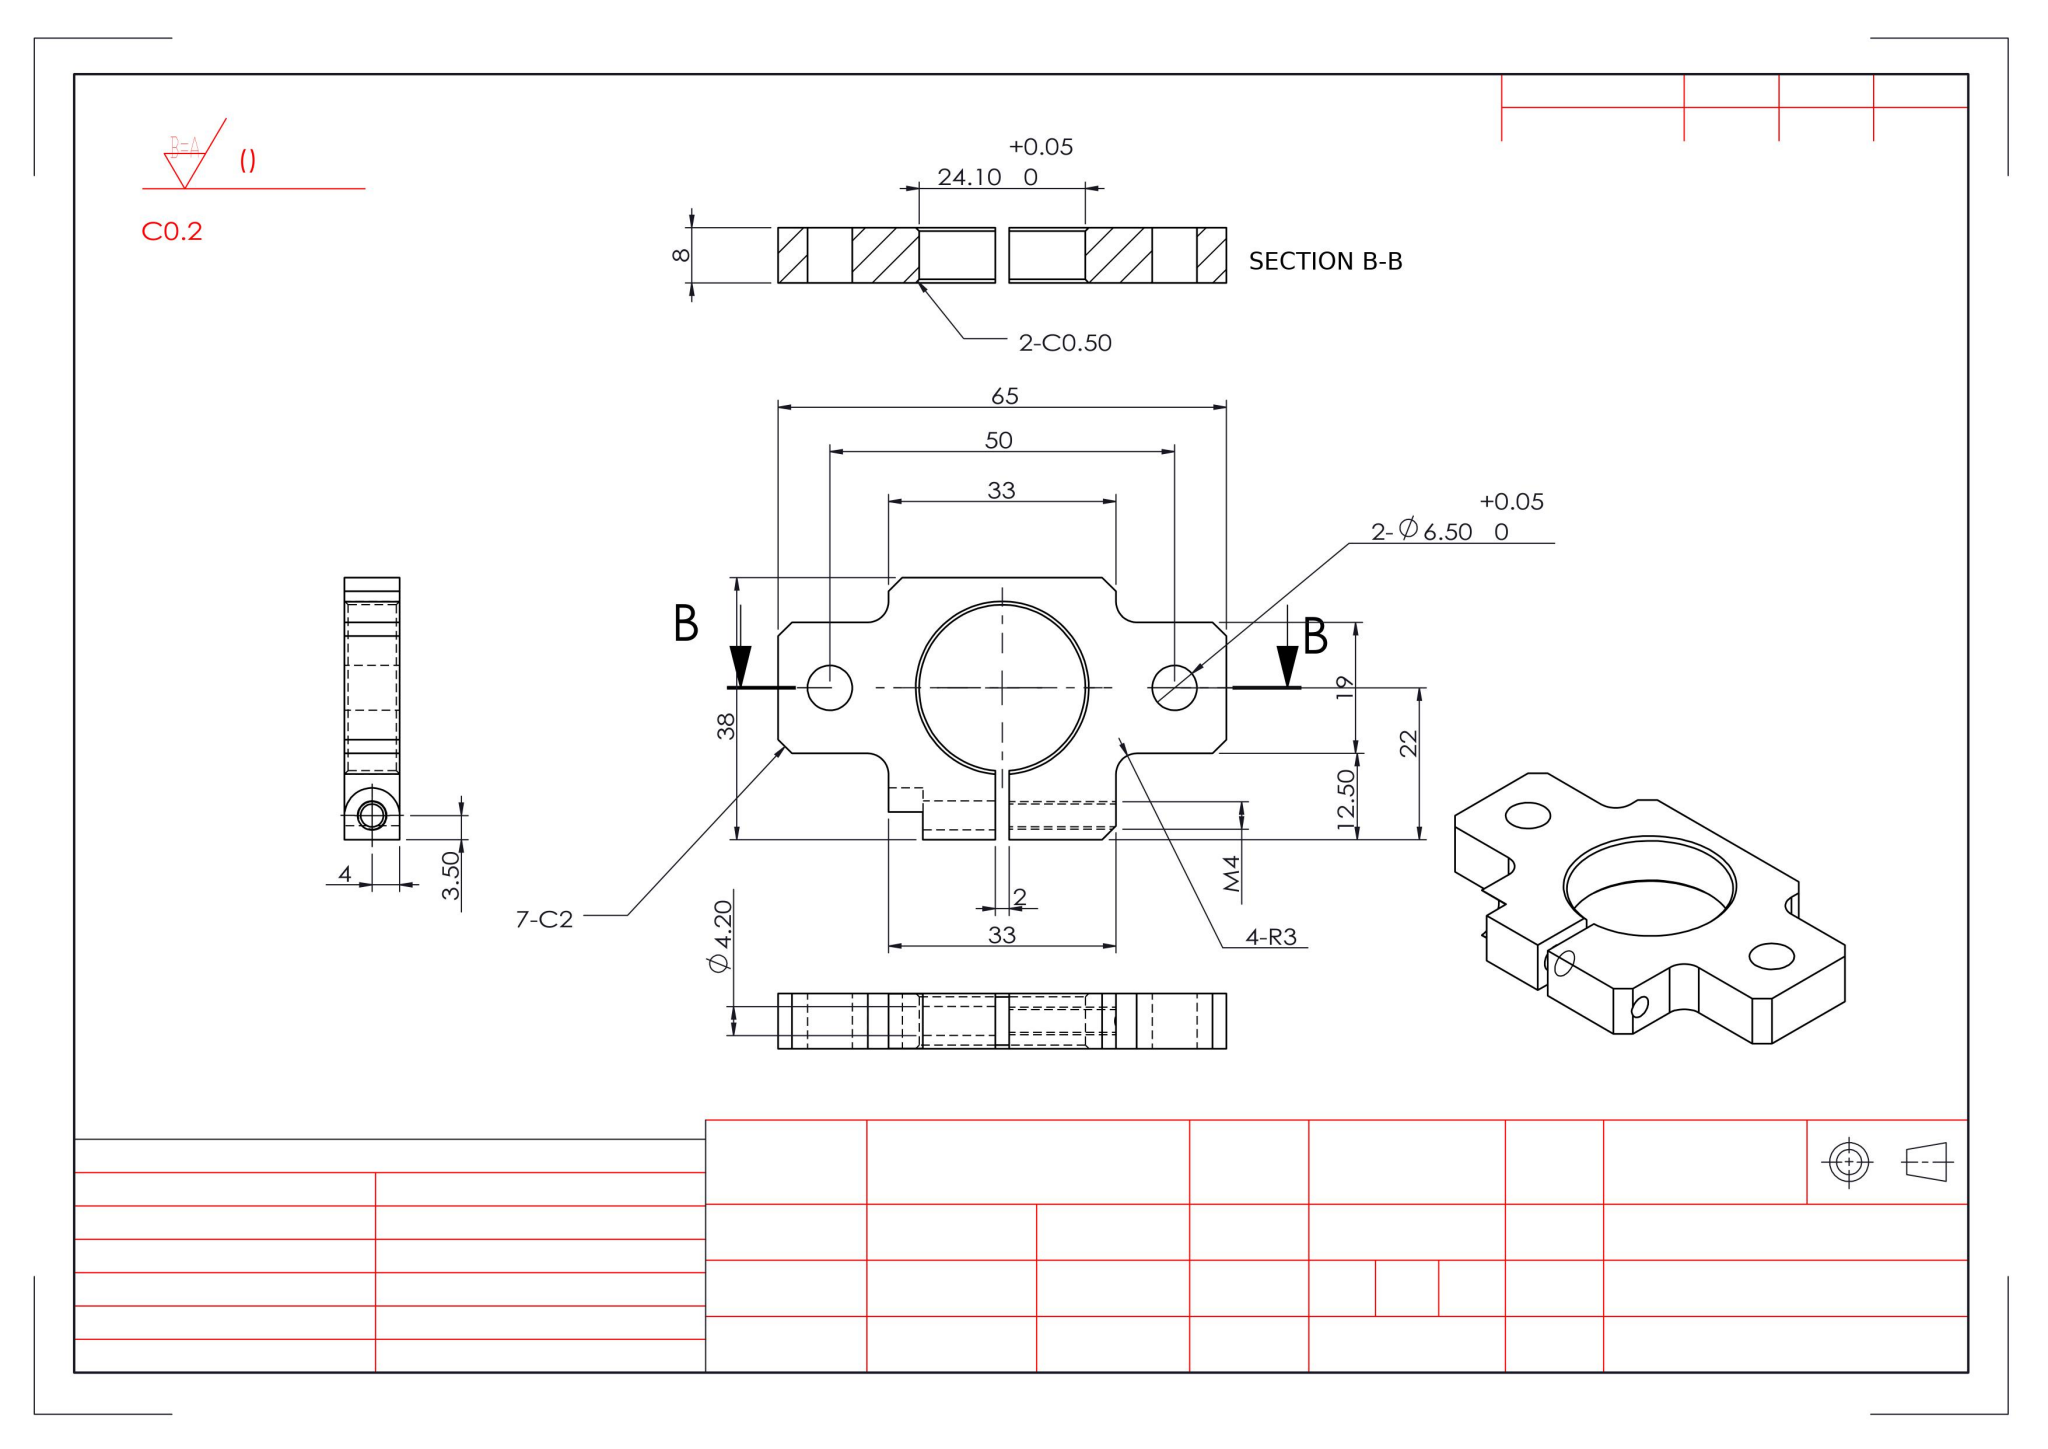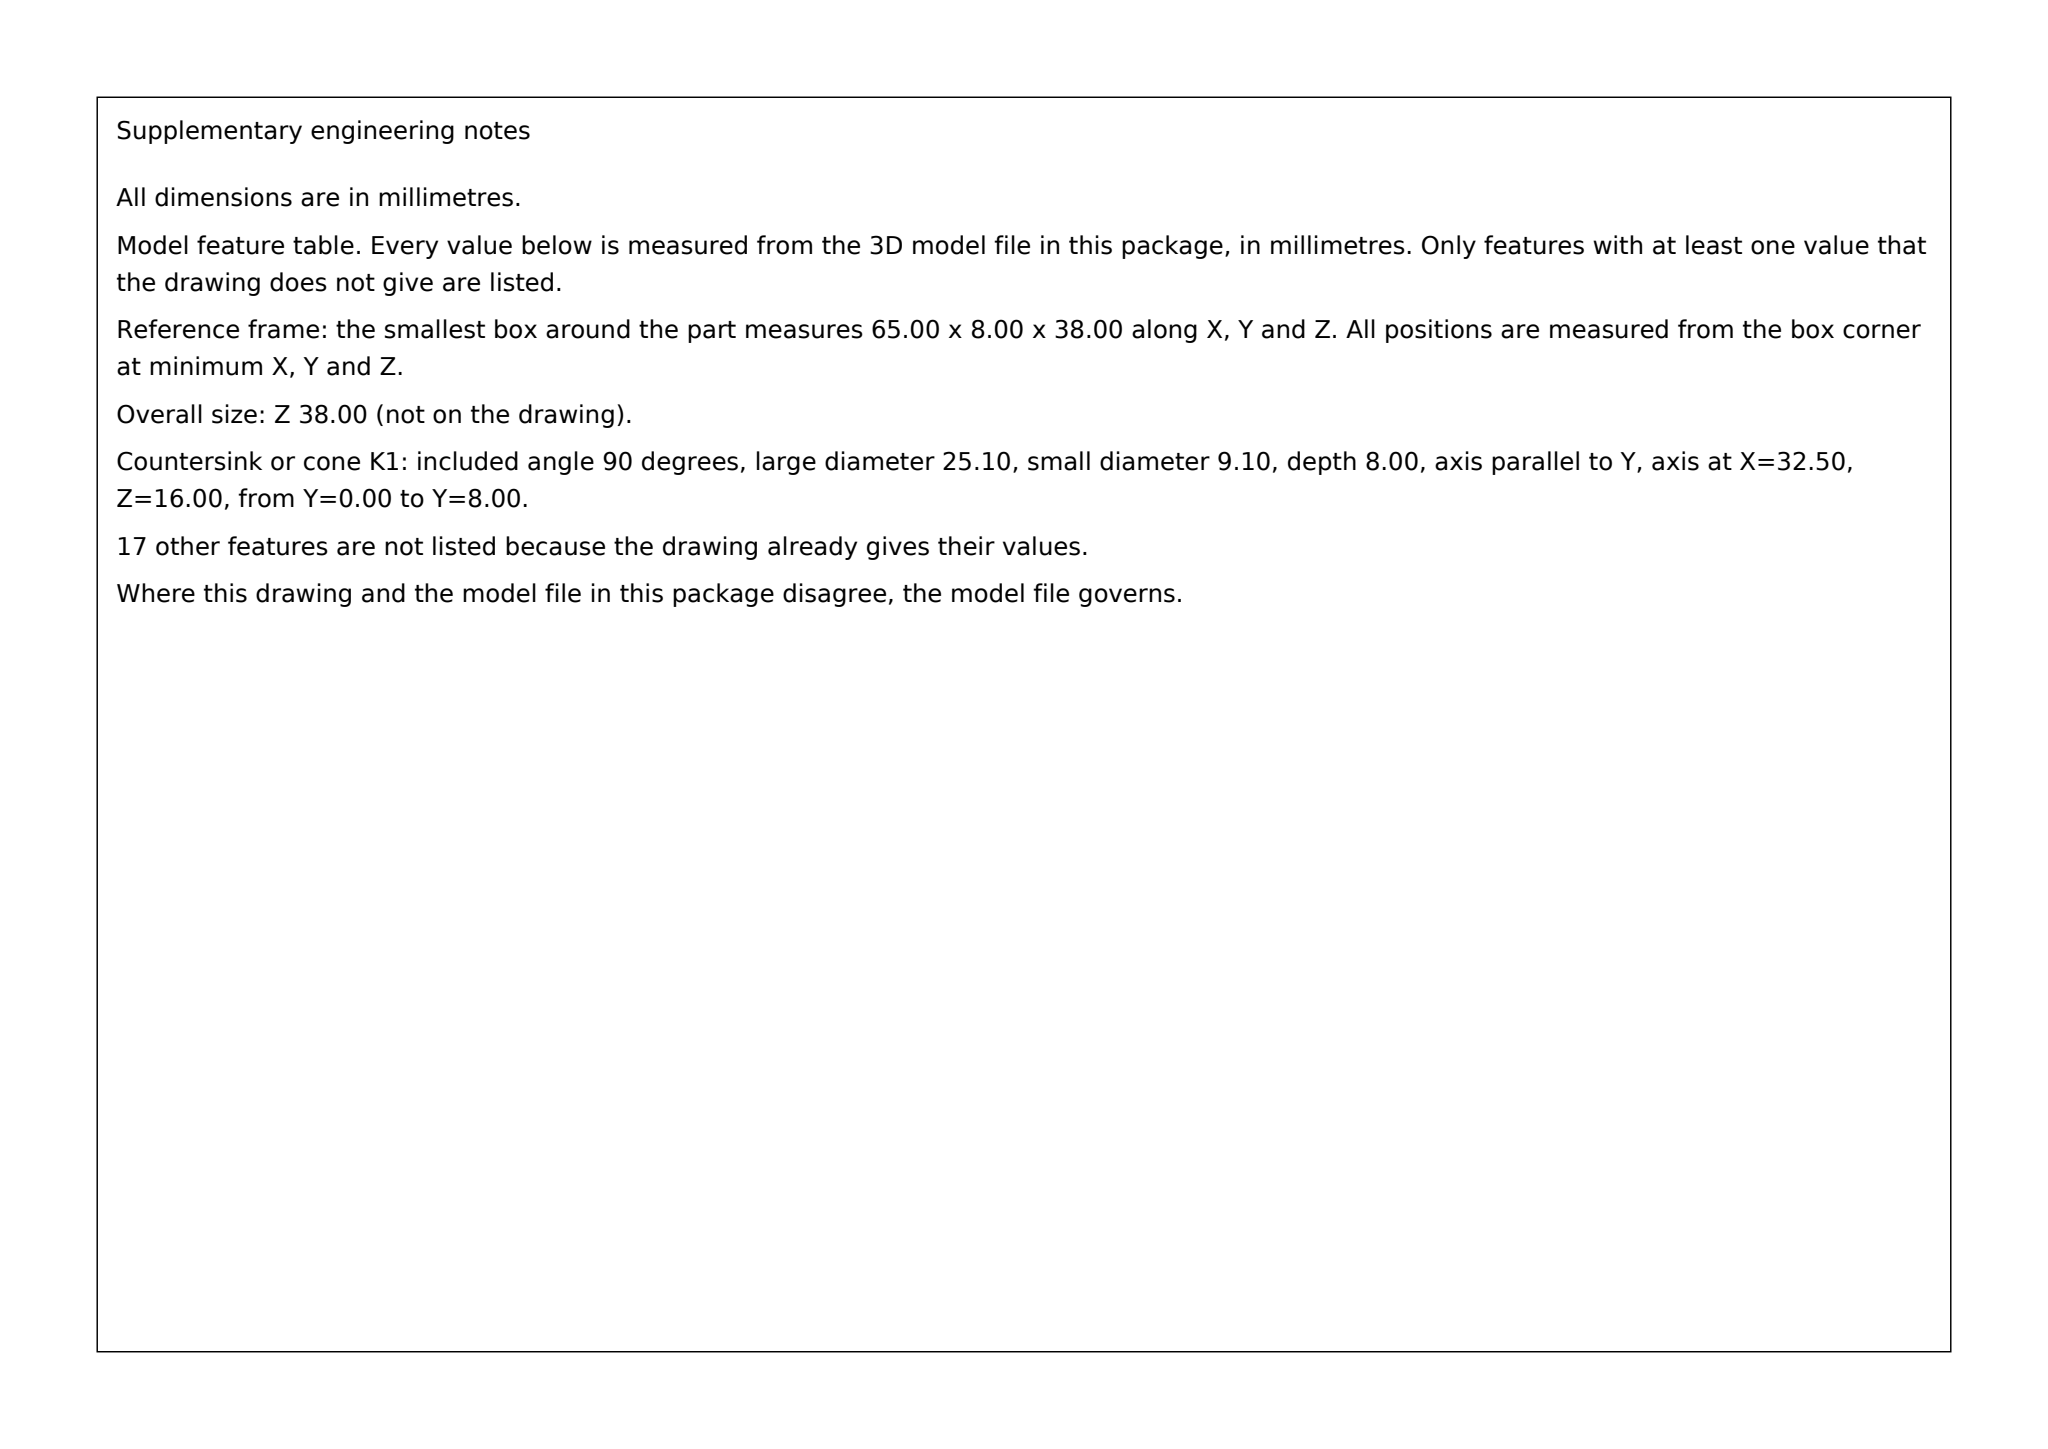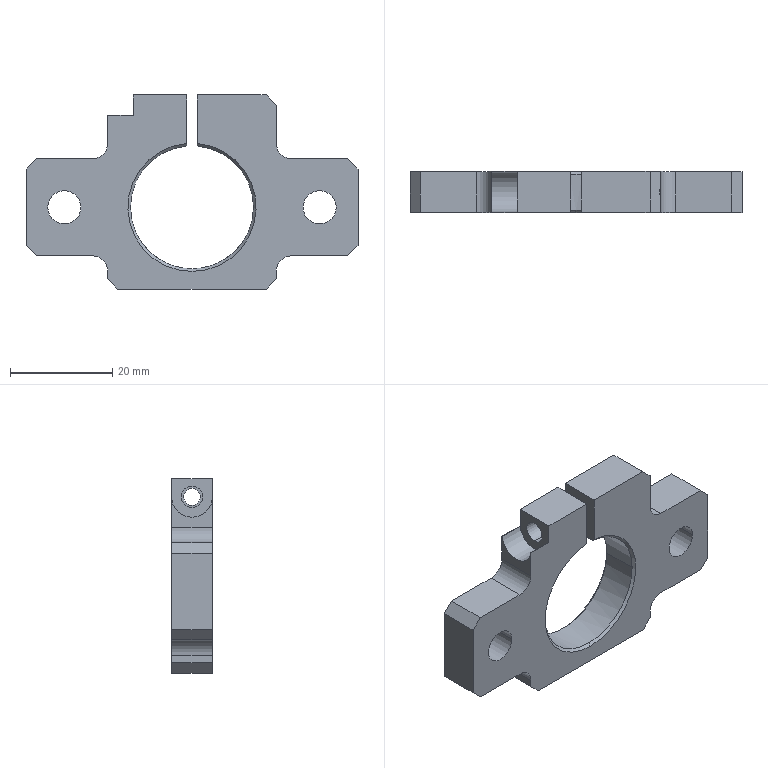Part | SolidWorks | mm | 1 solid | 46 faces | box 65 x 8 x 38 mm | volume 9944 mm3 | plane 27 | cylinder 16 | cone 3 | commonest cylinder face diameters 6.5 x4 6 x4 24.1 x3 3.3 x2 4.2 x2 7.99 x1